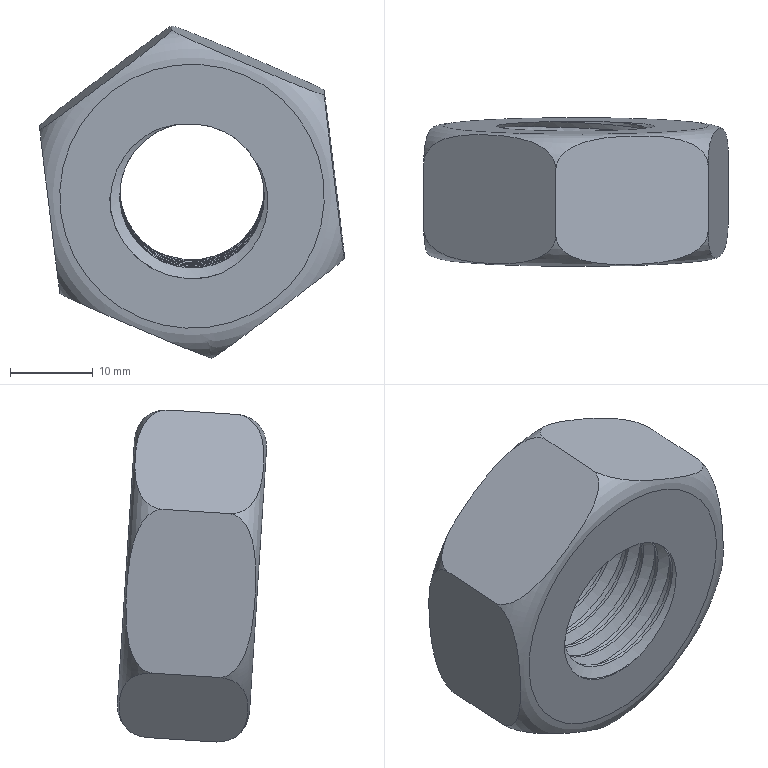Component | NX | CCJ-016 | 1 solid | 15 faces | volume 11974 mm3 | plane 9 | cylinder 2 | torus 2 | spline 2 | commonest cylinder face diameters 17.5 x1 20 x1